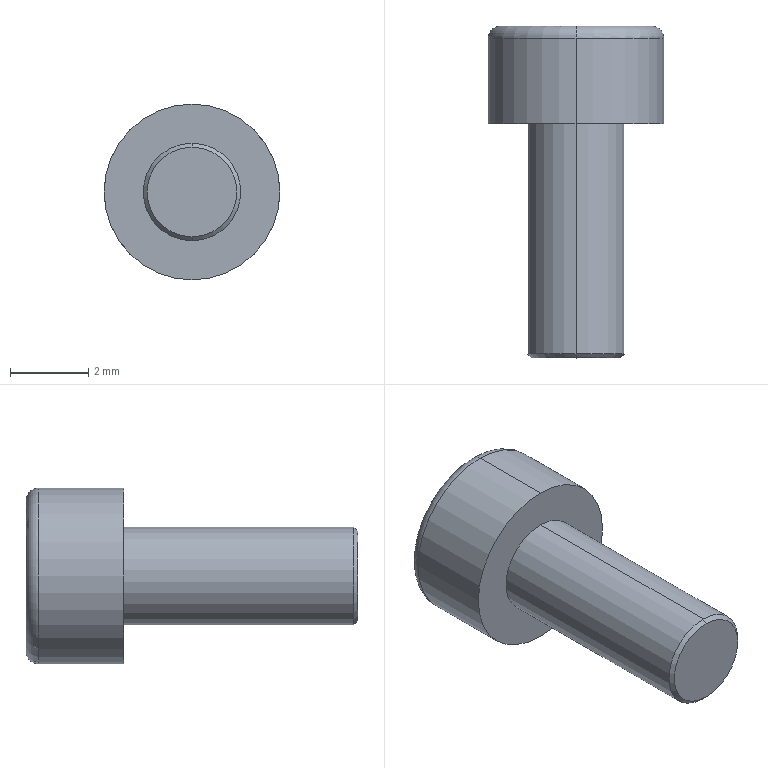Component | SolidWorks | hexagon socket head cap screws gb-1 | 1 solid | 25 faces | box 4.5 x 8.5 x 4.5 mm | volume 64 mm3 | plane 15 | cone 4 | cylinder 4 | torus 2 | commonest cylinder face diameters 2.5 x2 4.5 x2
STEP:
#1=COLOUR_RGB('',0.7922,0.8196,0.9333);
#2=FILL_AREA_STYLE_COLOUR('',#1);
#3=FILL_AREA_STYLE('',(#2));
#4=SURFACE_STYLE_FILL_AREA(#3);
#5=SURFACE_SIDE_STYLE('',(#4));
#6=SURFACE_STYLE_USAGE(.BOTH.,#5);
#7=PRESENTATION_STYLE_ASSIGNMENT((#6));
#8=CARTESIAN_POINT('',(-0.8485,0.2798,5.9));
#9=VERTEX_POINT('',#8);
#10=CARTESIAN_POINT('',(-0.8485,0.2798,5.991));
#11=VERTEX_POINT('',#10);
#12=CARTESIAN_POINT('',(-0.8485,0.2798,5.945));
#13=DIRECTION('',(0.,-1.,0.));
#14=DIRECTION('',(0.,0.,-1.));
#15=AXIS2_PLACEMENT_3D('',#12,#13,#14);
#16=CIRCLE('',#15,0.04528);
#17=EDGE_CURVE('',#9,#11,#16,.T.);
#18=ORIENTED_EDGE('',*,*,#17,.F.);
#19=CARTESIAN_POINT('',(-0.8485,0.2837,5.896));
#20=VERTEX_POINT('',#19);
#21=CARTESIAN_POINT('',(-0.8485,0.2798,5.9));
#22=DIRECTION('',(0.,0.7071,-0.7071));
#23=VECTOR('',#22,39.37);
#24=LINE('',#21,#23);
#25=EDGE_CURVE('',#9,#20,#24,.T.);
#26=ORIENTED_EDGE('',*,*,#25,.T.);
#27=CARTESIAN_POINT('',(-0.8485,0.2837,5.994));
#28=VERTEX_POINT('',#27);
#29=CARTESIAN_POINT('',(-0.8485,0.2837,5.945));
#30=DIRECTION('',(0.,1.,0.));
#31=DIRECTION('',(0.,0.,-1.));
#32=AXIS2_PLACEMENT_3D('',#29,#30,#31);
#33=CIRCLE('',#32,0.04921);
#34=EDGE_CURVE('',#28,#20,#33,.T.);
#35=ORIENTED_EDGE('',*,*,#34,.F.);
#36=CARTESIAN_POINT('',(-0.8485,0.2798,5.991));
#37=DIRECTION('',(0.,0.7071,0.7071));
#38=VECTOR('',#37,39.37);
#39=LINE('',#36,#38);
#40=EDGE_CURVE('',#11,#28,#39,.T.);
#41=ORIENTED_EDGE('',*,*,#40,.F.);
#42=EDGE_LOOP('',(#18,#26,#35,#41));
#43=FACE_OUTER_BOUND('',#42,.T.);
#44=CARTESIAN_POINT('',(-0.8485,0.2798,5.945));
#45=DIRECTION('',(0.,1.,0.));
#46=DIRECTION('',(0.,0.,1.));
#47=AXIS2_PLACEMENT_3D('',#44,#45,#46);
#48=CONICAL_SURFACE('',#47,0.04528,0.7854);
#49=ADVANCED_FACE('',(#43),#48,.T.);
#50=CARTESIAN_POINT('',(-0.8485,0.6144,6.022));
#51=VERTEX_POINT('',#50);
#52=CARTESIAN_POINT('',(-0.8485,0.6144,5.869));
#53=VERTEX_POINT('',#52);
#54=CARTESIAN_POINT('',(-0.8485,0.6144,5.945));
#55=DIRECTION('',(0.,1.,0.));
#56=DIRECTION('',(0.,0.,-1.));
#57=AXIS2_PLACEMENT_3D('',#54,#55,#56);
#58=CIRCLE('',#57,0.07628);
#59=EDGE_CURVE('',#51,#53,#58,.T.);
#60=ORIENTED_EDGE('',*,*,#59,.F.);
#61=CARTESIAN_POINT('',(-0.8485,0.6021,6.034));
#62=VERTEX_POINT('',#61);
#63=CARTESIAN_POINT('',(-0.8485,0.6021,6.022));
#64=DIRECTION('',(1.,0.,-0.));
#65=DIRECTION('',(0.,0.,-1.));
#66=AXIS2_PLACEMENT_3D('',#63,#64,#65);
#67=CIRCLE('',#66,0.0123);
#68=EDGE_CURVE('',#51,#62,#67,.T.);
#69=ORIENTED_EDGE('',*,*,#68,.T.);
#70=CARTESIAN_POINT('',(-0.8485,0.6021,5.857));
#71=VERTEX_POINT('',#70);
#72=CARTESIAN_POINT('',(-0.8485,0.6021,5.945));
#73=DIRECTION('',(0.,-1.,0.));
#74=DIRECTION('',(0.,0.,-1.));
#75=AXIS2_PLACEMENT_3D('',#72,#73,#74);
#76=CIRCLE('',#75,0.08858);
#77=EDGE_CURVE('',#71,#62,#76,.T.);
#78=ORIENTED_EDGE('',*,*,#77,.F.);
#79=CARTESIAN_POINT('',(-0.8485,0.6021,5.869));
#80=DIRECTION('',(-1.,0.,0.));
#81=DIRECTION('',(0.,0.,1.));
#82=AXIS2_PLACEMENT_3D('',#79,#80,#81);
#83=CIRCLE('',#82,0.0123);
#84=EDGE_CURVE('',#53,#71,#83,.T.);
#85=ORIENTED_EDGE('',*,*,#84,.F.);
#86=EDGE_LOOP('',(#60,#69,#78,#85));
#87=FACE_OUTER_BOUND('',#86,.T.);
#88=CARTESIAN_POINT('',(-0.8485,0.6021,5.945));
#89=DIRECTION('',(0.,-1.,0.));
#90=DIRECTION('',(0.,0.,-1.));
#91=AXIS2_PLACEMENT_3D('',#88,#89,#90);
#92=TOROIDAL_SURFACE('',#91,0.07628,0.0123);
#93=ADVANCED_FACE('',(#87),#92,.T.);
#94=CARTESIAN_POINT('',(-0.8485,0.5484,5.945));
#95=VERTEX_POINT('',#94);
#96=CARTESIAN_POINT('',(-0.8485,0.5711,5.985));
#97=VERTEX_POINT('',#96);
#98=CARTESIAN_POINT('',(-0.8485,0.5711,5.985));
#99=DIRECTION('',(0.,0.5,0.866));
#100=VECTOR('',#99,39.37);
#101=LINE('',#98,#100);
#102=EDGE_CURVE('',#95,#97,#101,.T.);
#103=ORIENTED_EDGE('',*,*,#102,.F.);
#104=CARTESIAN_POINT('',(-0.8485,0.5711,5.906));
#105=VERTEX_POINT('',#104);
#106=CARTESIAN_POINT('',(-0.8485,0.5711,5.906));
#107=DIRECTION('',(0.,0.5,-0.866));
#108=VECTOR('',#107,39.37);
#109=LINE('',#106,#108);
#110=EDGE_CURVE('',#95,#105,#109,.T.);
#111=ORIENTED_EDGE('',*,*,#110,.T.);
#112=CARTESIAN_POINT('',(-0.8682,0.5711,5.911));
#113=VERTEX_POINT('',#112);
#114=CARTESIAN_POINT('',(-0.8485,0.5711,5.945));
#115=DIRECTION('',(0.,1.,0.));
#116=DIRECTION('',(0.,0.,-1.));
#117=AXIS2_PLACEMENT_3D('',#114,#115,#116);
#118=CIRCLE('',#117,0.03937);
#119=EDGE_CURVE('',#105,#113,#118,.T.);
#120=ORIENTED_EDGE('',*,*,#119,.T.);
#121=CARTESIAN_POINT('',(-0.8879,0.5711,5.945));
#122=VERTEX_POINT('',#121);
#123=CARTESIAN_POINT('',(-0.8485,0.5711,5.945));
#124=DIRECTION('',(0.,1.,0.));
#125=DIRECTION('',(0.,0.,-1.));
#126=AXIS2_PLACEMENT_3D('',#123,#124,#125);
#127=CIRCLE('',#126,0.03937);
#128=EDGE_CURVE('',#113,#122,#127,.T.);
#129=ORIENTED_EDGE('',*,*,#128,.T.);
#130=CARTESIAN_POINT('',(-0.8682,0.5711,5.979));
#131=VERTEX_POINT('',#130);
#132=CARTESIAN_POINT('',(-0.8485,0.5711,5.945));
#133=DIRECTION('',(0.,1.,0.));
#134=DIRECTION('',(-0.,0.,-1.));
#135=AXIS2_PLACEMENT_3D('',#132,#133,#134);
#136=CIRCLE('',#135,0.03937);
#137=EDGE_CURVE('',#122,#131,#136,.T.);
#138=ORIENTED_EDGE('',*,*,#137,.T.);
#139=CARTESIAN_POINT('',(-0.8485,0.5711,5.945));
#140=DIRECTION('',(0.,1.,0.));
#141=DIRECTION('',(0.,0.,-1.));
#142=AXIS2_PLACEMENT_3D('',#139,#140,#141);
#143=CIRCLE('',#142,0.03937);
#144=EDGE_CURVE('',#131,#97,#143,.T.);
#145=ORIENTED_EDGE('',*,*,#144,.T.);
#146=EDGE_LOOP('',(#103,#111,#120,#129,#138,#145));
#147=FACE_OUTER_BOUND('',#146,.T.);
#148=CARTESIAN_POINT('',(-0.8485,0.5711,5.945));
#149=DIRECTION('',(0.,1.,0.));
#150=DIRECTION('',(0.,0.,1.));
#151=AXIS2_PLACEMENT_3D('',#148,#149,#150);
#152=CONICAL_SURFACE('',#151,0.03937,1.047);
#153=ADVANCED_FACE('',(#147),#152,.F.);
#154=ORIENTED_EDGE('',*,*,#34,.T.);
#155=CARTESIAN_POINT('',(-0.8485,0.516,5.896));
#156=VERTEX_POINT('',#155);
#157=CARTESIAN_POINT('',(-0.8485,0.2798,5.896));
#158=DIRECTION('',(0.,1.,0.));
#159=VECTOR('',#158,39.37);
#160=LINE('',#157,#159);
#161=EDGE_CURVE('',#20,#156,#160,.T.);
#162=ORIENTED_EDGE('',*,*,#161,.T.);
#163=CARTESIAN_POINT('',(-0.8485,0.516,5.994));
#164=VERTEX_POINT('',#163);
#165=CARTESIAN_POINT('',(-0.8485,0.516,5.945));
#166=DIRECTION('',(0.,-1.,0.));
#167=DIRECTION('',(0.,0.,-1.));
#168=AXIS2_PLACEMENT_3D('',#165,#166,#167);
#169=CIRCLE('',#168,0.04921);
#170=EDGE_CURVE('',#156,#164,#169,.T.);
#171=ORIENTED_EDGE('',*,*,#170,.T.);
#172=CARTESIAN_POINT('',(-0.8485,0.2798,5.994));
#173=DIRECTION('',(0.,1.,0.));
#174=VECTOR('',#173,39.37);
#175=LINE('',#172,#174);
#176=EDGE_CURVE('',#28,#164,#175,.T.);
#177=ORIENTED_EDGE('',*,*,#176,.F.);
#178=EDGE_LOOP('',(#154,#162,#171,#177));
#179=FACE_OUTER_BOUND('',#178,.T.);
#180=CARTESIAN_POINT('',(-0.8485,0.2798,5.945));
#181=DIRECTION('',(0.,1.,0.));
#182=DIRECTION('',(0.,0.,1.));
#183=AXIS2_PLACEMENT_3D('',#180,#181,#182);
#184=CYLINDRICAL_SURFACE('',#183,0.04921);
#185=ADVANCED_FACE('',(#179),#184,.T.);
#186=CARTESIAN_POINT('',(-0.8485,0.516,5.857));
#187=VERTEX_POINT('',#186);
#188=CARTESIAN_POINT('',(-0.8485,0.516,6.034));
#189=VERTEX_POINT('',#188);
#190=CARTESIAN_POINT('',(-0.8485,0.516,5.945));
#191=DIRECTION('',(0.,-1.,0.));
#192=DIRECTION('',(0.,0.,-1.));
#193=AXIS2_PLACEMENT_3D('',#190,#191,#192);
#194=CIRCLE('',#193,0.08858);
#195=EDGE_CURVE('',#187,#189,#194,.T.);
#196=ORIENTED_EDGE('',*,*,#195,.F.);
#197=CARTESIAN_POINT('',(-0.8485,0.516,5.857));
#198=DIRECTION('',(0.,1.,0.));
#199=VECTOR('',#198,39.37);
#200=LINE('',#197,#199);
#201=EDGE_CURVE('',#187,#71,#200,.T.);
#202=ORIENTED_EDGE('',*,*,#201,.T.);
#203=ORIENTED_EDGE('',*,*,#77,.T.);
#204=CARTESIAN_POINT('',(-0.8485,0.516,6.034));
#205=DIRECTION('',(0.,1.,0.));
#206=VECTOR('',#205,39.37);
#207=LINE('',#204,#206);
#208=EDGE_CURVE('',#189,#62,#207,.T.);
#209=ORIENTED_EDGE('',*,*,#208,.F.);
#210=EDGE_LOOP('',(#196,#202,#203,#209));
#211=FACE_OUTER_BOUND('',#210,.T.);
#212=CARTESIAN_POINT('',(-0.8485,0.516,5.945));
#213=DIRECTION('',(0.,1.,0.));
#214=DIRECTION('',(0.,0.,1.));
#215=AXIS2_PLACEMENT_3D('',#212,#213,#214);
#216=CYLINDRICAL_SURFACE('',#215,0.08858);
#217=ADVANCED_FACE('',(#211),#216,.T.);
#218=ORIENTED_EDGE('',*,*,#128,.F.);
#219=CARTESIAN_POINT('',(-0.8879,0.5711,5.923));
#220=VERTEX_POINT('',#219);
#221=CARTESIAN_POINT('',(-0.8879,0.5711,5.923));
#222=DIRECTION('',(0.866,0.,-0.5));
#223=VECTOR('',#222,39.37);
#224=LINE('',#221,#223);
#225=EDGE_CURVE('',#220,#113,#224,.T.);
#226=ORIENTED_EDGE('',*,*,#225,.F.);
#227=CARTESIAN_POINT('',(-0.8879,0.5711,5.968));
#228=DIRECTION('',(0.,0.,-1.));
#229=VECTOR('',#228,39.37);
#230=LINE('',#227,#229);
#231=EDGE_CURVE('',#122,#220,#230,.T.);
#232=ORIENTED_EDGE('',*,*,#231,.F.);
#233=EDGE_LOOP('',(#218,#226,#232));
#234=FACE_OUTER_BOUND('',#233,.T.);
#235=CARTESIAN_POINT('',(-0.8485,0.5711,5.9));
#236=DIRECTION('',(0.,-1.,0.));
#237=DIRECTION('',(0.,0.,-1.));
#238=AXIS2_PLACEMENT_3D('',#235,#236,#237);
#239=PLANE('',#238);
#240=ADVANCED_FACE('',(#234),#239,.F.);
#241=ORIENTED_EDGE('',*,*,#137,.F.);
#242=CARTESIAN_POINT('',(-0.8879,0.5711,5.968));
#243=VERTEX_POINT('',#242);
#244=CARTESIAN_POINT('',(-0.8879,0.5711,5.968));
#245=DIRECTION('',(0.,0.,-1.));
#246=VECTOR('',#245,39.37);
#247=LINE('',#244,#246);
#248=EDGE_CURVE('',#243,#122,#247,.T.);
#249=ORIENTED_EDGE('',*,*,#248,.F.);
#250=CARTESIAN_POINT('',(-0.8485,0.5711,5.991));
#251=DIRECTION('',(-0.866,0.,-0.5));
#252=VECTOR('',#251,39.37);
#253=LINE('',#250,#252);
#254=EDGE_CURVE('',#131,#243,#253,.T.);
#255=ORIENTED_EDGE('',*,*,#254,.F.);
#256=EDGE_LOOP('',(#241,#249,#255));
#257=FACE_OUTER_BOUND('',#256,.T.);
#258=CARTESIAN_POINT('',(-0.8485,0.5711,5.9));
#259=DIRECTION('',(0.,-1.,0.));
#260=DIRECTION('',(0.,0.,-1.));
#261=AXIS2_PLACEMENT_3D('',#258,#259,#260);
#262=PLANE('',#261);
#263=ADVANCED_FACE('',(#257),#262,.F.);
#264=ORIENTED_EDGE('',*,*,#144,.F.);
#265=CARTESIAN_POINT('',(-0.8485,0.5711,5.991));
#266=VERTEX_POINT('',#265);
#267=CARTESIAN_POINT('',(-0.8485,0.5711,5.991));
#268=DIRECTION('',(-0.866,0.,-0.5));
#269=VECTOR('',#268,39.37);
#270=LINE('',#267,#269);
#271=EDGE_CURVE('',#266,#131,#270,.T.);
#272=ORIENTED_EDGE('',*,*,#271,.F.);
#273=CARTESIAN_POINT('',(-0.8288,0.5711,5.979));
#274=VERTEX_POINT('',#273);
#275=CARTESIAN_POINT('',(-0.8092,0.5711,5.968));
#276=DIRECTION('',(-0.866,0.,0.5));
#277=VECTOR('',#276,39.37);
#278=LINE('',#275,#277);
#279=EDGE_CURVE('',#274,#266,#278,.T.);
#280=ORIENTED_EDGE('',*,*,#279,.F.);
#281=CARTESIAN_POINT('',(-0.8485,0.5711,5.945));
#282=DIRECTION('',(0.,1.,0.));
#283=DIRECTION('',(0.,0.,-1.));
#284=AXIS2_PLACEMENT_3D('',#281,#282,#283);
#285=CIRCLE('',#284,0.03937);
#286=EDGE_CURVE('',#97,#274,#285,.T.);
#287=ORIENTED_EDGE('',*,*,#286,.F.);
#288=EDGE_LOOP('',(#264,#272,#280,#287));
#289=FACE_OUTER_BOUND('',#288,.T.);
#290=CARTESIAN_POINT('',(-0.8485,0.5711,5.9));
#291=DIRECTION('',(0.,-1.,0.));
#292=DIRECTION('',(0.,0.,-1.));
#293=AXIS2_PLACEMENT_3D('',#290,#291,#292);
#294=PLANE('',#293);
#295=ADVANCED_FACE('',(#289),#294,.F.);
#296=CARTESIAN_POINT('',(-0.8092,0.5711,5.945));
#297=VERTEX_POINT('',#296);
#298=CARTESIAN_POINT('',(-0.8485,0.5711,5.945));
#299=DIRECTION('',(0.,1.,0.));
#300=DIRECTION('',(0.,0.,-1.));
#301=AXIS2_PLACEMENT_3D('',#298,#299,#300);
#302=CIRCLE('',#301,0.03937);
#303=EDGE_CURVE('',#274,#297,#302,.T.);
#304=ORIENTED_EDGE('',*,*,#303,.F.);
#305=CARTESIAN_POINT('',(-0.8092,0.5711,5.968));
#306=VERTEX_POINT('',#305);
#307=CARTESIAN_POINT('',(-0.8092,0.5711,5.968));
#308=DIRECTION('',(-0.866,0.,0.5));
#309=VECTOR('',#308,39.37);
#310=LINE('',#307,#309);
#311=EDGE_CURVE('',#306,#274,#310,.T.);
#312=ORIENTED_EDGE('',*,*,#311,.F.);
#313=CARTESIAN_POINT('',(-0.8092,0.5711,5.923));
#314=DIRECTION('',(0.,0.,1.));
#315=VECTOR('',#314,39.37);
#316=LINE('',#313,#315);
#317=EDGE_CURVE('',#297,#306,#316,.T.);
#318=ORIENTED_EDGE('',*,*,#317,.F.);
#319=EDGE_LOOP('',(#304,#312,#318));
#320=FACE_OUTER_BOUND('',#319,.T.);
#321=CARTESIAN_POINT('',(-0.8485,0.5711,5.9));
#322=DIRECTION('',(0.,-1.,0.));
#323=DIRECTION('',(0.,0.,-1.));
#324=AXIS2_PLACEMENT_3D('',#321,#322,#323);
#325=PLANE('',#324);
#326=ADVANCED_FACE('',(#320),#325,.F.);
#327=CARTESIAN_POINT('',(-0.8288,0.5711,5.911));
#328=VERTEX_POINT('',#327);
#329=CARTESIAN_POINT('',(-0.8485,0.5711,5.945));
#330=DIRECTION('',(0.,-1.,0.));
#331=DIRECTION('',(0.,0.,-1.));
#332=AXIS2_PLACEMENT_3D('',#329,#330,#331);
#333=CIRCLE('',#332,0.03937);
#334=EDGE_CURVE('',#328,#297,#333,.T.);
#335=ORIENTED_EDGE('',*,*,#334,.T.);
#336=CARTESIAN_POINT('',(-0.8092,0.5711,5.923));
#337=VERTEX_POINT('',#336);
#338=CARTESIAN_POINT('',(-0.8092,0.5711,5.923));
#339=DIRECTION('',(0.,0.,1.));
#340=VECTOR('',#339,39.37);
#341=LINE('',#338,#340);
#342=EDGE_CURVE('',#337,#297,#341,.T.);
#343=ORIENTED_EDGE('',*,*,#342,.F.);
#344=CARTESIAN_POINT('',(-0.8485,0.5711,5.9));
#345=DIRECTION('',(0.866,0.,0.5));
#346=VECTOR('',#345,39.37);
#347=LINE('',#344,#346);
#348=EDGE_CURVE('',#328,#337,#347,.T.);
#349=ORIENTED_EDGE('',*,*,#348,.F.);
#350=EDGE_LOOP('',(#335,#343,#349));
#351=FACE_OUTER_BOUND('',#350,.T.);
#352=CARTESIAN_POINT('',(-0.8485,0.5711,5.9));
#353=DIRECTION('',(0.,-1.,0.));
#354=DIRECTION('',(0.,0.,-1.));
#355=AXIS2_PLACEMENT_3D('',#352,#353,#354);
#356=PLANE('',#355);
#357=ADVANCED_FACE('',(#351),#356,.F.);
#358=CARTESIAN_POINT('',(-0.8485,0.5711,5.945));
#359=DIRECTION('',(0.,1.,0.));
#360=DIRECTION('',(-0.,0.,-1.));
#361=AXIS2_PLACEMENT_3D('',#358,#359,#360);
#362=CIRCLE('',#361,0.03937);
#363=EDGE_CURVE('',#328,#105,#362,.T.);
#364=ORIENTED_EDGE('',*,*,#363,.F.);
#365=CARTESIAN_POINT('',(-0.8485,0.5711,5.9));
#366=VERTEX_POINT('',#365);
#367=CARTESIAN_POINT('',(-0.8485,0.5711,5.9));
#368=DIRECTION('',(0.866,0.,0.5));
#369=VECTOR('',#368,39.37);
#370=LINE('',#367,#369);
#371=EDGE_CURVE('',#366,#328,#370,.T.);
#372=ORIENTED_EDGE('',*,*,#371,.F.);
#373=CARTESIAN_POINT('',(-0.8879,0.5711,5.923));
#374=DIRECTION('',(0.866,0.,-0.5));
#375=VECTOR('',#374,39.37);
#376=LINE('',#373,#375);
#377=EDGE_CURVE('',#113,#366,#376,.T.);
#378=ORIENTED_EDGE('',*,*,#377,.F.);
#379=ORIENTED_EDGE('',*,*,#119,.F.);
#380=EDGE_LOOP('',(#364,#372,#378,#379));
#381=FACE_OUTER_BOUND('',#380,.T.);
#382=CARTESIAN_POINT('',(-0.8485,0.5711,5.9));
#383=DIRECTION('',(0.,-1.,0.));
#384=DIRECTION('',(0.,0.,-1.));
#385=AXIS2_PLACEMENT_3D('',#382,#383,#384);
#386=PLANE('',#385);
#387=ADVANCED_FACE('',(#381),#386,.F.);
#388=CARTESIAN_POINT('',(-0.8485,0.6144,5.945));
#389=DIRECTION('',(0.,1.,0.));
#390=DIRECTION('',(0.,0.,-1.));
#391=AXIS2_PLACEMENT_3D('',#388,#389,#390);
#392=CIRCLE('',#391,0.07628);
#393=EDGE_CURVE('',#53,#51,#392,.T.);
#394=ORIENTED_EDGE('',*,*,#393,.T.);
#395=ORIENTED_EDGE('',*,*,#59,.T.);
#396=EDGE_LOOP('',(#394,#395));
#397=FACE_OUTER_BOUND('',#396,.T.);
#398=CARTESIAN_POINT('',(-0.8879,0.6144,5.923));
#399=VERTEX_POINT('',#398);
#400=CARTESIAN_POINT('',(-0.8485,0.6144,5.9));
#401=VERTEX_POINT('',#400);
#402=CARTESIAN_POINT('',(-0.8879,0.6144,5.923));
#403=DIRECTION('',(0.866,0.,-0.5));
#404=VECTOR('',#403,39.37);
#405=LINE('',#402,#404);
#406=EDGE_CURVE('',#399,#401,#405,.T.);
#407=ORIENTED_EDGE('',*,*,#406,.T.);
#408=CARTESIAN_POINT('',(-0.8092,0.6144,5.923));
#409=VERTEX_POINT('',#408);
#410=CARTESIAN_POINT('',(-0.8485,0.6144,5.9));
#411=DIRECTION('',(0.866,0.,0.5));
#412=VECTOR('',#411,39.37);
#413=LINE('',#410,#412);
#414=EDGE_CURVE('',#401,#409,#413,.T.);
#415=ORIENTED_EDGE('',*,*,#414,.T.);
#416=CARTESIAN_POINT('',(-0.8092,0.6144,5.968));
#417=VERTEX_POINT('',#416);
#418=CARTESIAN_POINT('',(-0.8092,0.6144,5.923));
#419=DIRECTION('',(0.,0.,1.));
#420=VECTOR('',#419,39.37);
#421=LINE('',#418,#420);
#422=EDGE_CURVE('',#409,#417,#421,.T.);
#423=ORIENTED_EDGE('',*,*,#422,.T.);
#424=CARTESIAN_POINT('',(-0.8485,0.6144,5.991));
#425=VERTEX_POINT('',#424);
#426=CARTESIAN_POINT('',(-0.8092,0.6144,5.968));
#427=DIRECTION('',(-0.866,0.,0.5));
#428=VECTOR('',#427,39.37);
#429=LINE('',#426,#428);
#430=EDGE_CURVE('',#417,#425,#429,.T.);
#431=ORIENTED_EDGE('',*,*,#430,.T.);
#432=CARTESIAN_POINT('',(-0.8879,0.6144,5.968));
#433=VERTEX_POINT('',#432);
#434=CARTESIAN_POINT('',(-0.8485,0.6144,5.991));
#435=DIRECTION('',(-0.866,0.,-0.5));
#436=VECTOR('',#435,39.37);
#437=LINE('',#434,#436);
#438=EDGE_CURVE('',#425,#433,#437,.T.);
#439=ORIENTED_EDGE('',*,*,#438,.T.);
#440=CARTESIAN_POINT('',(-0.8879,0.6144,5.968));
#441=DIRECTION('',(0.,0.,-1.));
#442=VECTOR('',#441,39.37);
#443=LINE('',#440,#442);
#444=EDGE_CURVE('',#433,#399,#443,.T.);
#445=ORIENTED_EDGE('',*,*,#444,.T.);
#446=EDGE_LOOP('',(#407,#415,#423,#431,#439,#445));
#447=FACE_BOUND('',#446,.T.);
#448=CARTESIAN_POINT('',(-0.8485,0.6144,5.945));
#449=DIRECTION('',(0.,-1.,0.));
#450=DIRECTION('',(0.,0.,-1.));
#451=AXIS2_PLACEMENT_3D('',#448,#449,#450);
#452=PLANE('',#451);
#453=ADVANCED_FACE('',(#397,#447),#452,.F.);
#454=CARTESIAN_POINT('',(-0.8485,0.516,5.945));
#455=DIRECTION('',(0.,-1.,0.));
#456=DIRECTION('',(0.,0.,-1.));
#457=AXIS2_PLACEMENT_3D('',#454,#455,#456);
#458=CIRCLE('',#457,0.08858);
#459=EDGE_CURVE('',#189,#187,#458,.T.);
#460=ORIENTED_EDGE('',*,*,#459,.T.);
#461=ORIENTED_EDGE('',*,*,#195,.T.);
#462=EDGE_LOOP('',(#460,#461));
#463=FACE_OUTER_BOUND('',#462,.T.);
#464=CARTESIAN_POINT('',(-0.8485,0.516,5.945));
#465=DIRECTION('',(0.,-1.,0.));
#466=DIRECTION('',(0.,0.,-1.));
#467=AXIS2_PLACEMENT_3D('',#464,#465,#466);
#468=CIRCLE('',#467,0.04921);
#469=EDGE_CURVE('',#164,#156,#468,.T.);
#470=ORIENTED_EDGE('',*,*,#469,.F.);
#471=ORIENTED_EDGE('',*,*,#170,.F.);
#472=EDGE_LOOP('',(#470,#471));
#473=FACE_BOUND('',#472,.T.);
#474=CARTESIAN_POINT('',(-0.8485,0.516,5.945));
#475=DIRECTION('',(0.,-1.,0.));
#476=DIRECTION('',(0.,0.,-1.));
#477=AXIS2_PLACEMENT_3D('',#474,#475,#476);
#478=PLANE('',#477);
#479=ADVANCED_FACE('',(#463,#473),#478,.T.);
#480=ORIENTED_EDGE('',*,*,#201,.F.);
#481=ORIENTED_EDGE('',*,*,#459,.F.);
#482=ORIENTED_EDGE('',*,*,#208,.T.);
#483=CARTESIAN_POINT('',(-0.8485,0.6021,5.945));
#484=DIRECTION('',(0.,-1.,0.));
#485=DIRECTION('',(0.,0.,-1.));
#486=AXIS2_PLACEMENT_3D('',#483,#484,#485);
#487=CIRCLE('',#486,0.08858);
#488=EDGE_CURVE('',#62,#71,#487,.T.);
#489=ORIENTED_EDGE('',*,*,#488,.T.);
#490=EDGE_LOOP('',(#480,#481,#482,#489));
#491=FACE_OUTER_BOUND('',#490,.T.);
#492=CARTESIAN_POINT('',(-0.8485,0.516,5.945));
#493=DIRECTION('',(0.,1.,0.));
#494=DIRECTION('',(0.,0.,1.));
#495=AXIS2_PLACEMENT_3D('',#492,#493,#494);
#496=CYLINDRICAL_SURFACE('',#495,0.08858);
#497=ADVANCED_FACE('',(#491),#496,.T.);
#498=ORIENTED_EDGE('',*,*,#161,.F.);
#499=CARTESIAN_POINT('',(-0.8485,0.2837,5.945));
#500=DIRECTION('',(0.,1.,0.));
#501=DIRECTION('',(0.,0.,-1.));
#502=AXIS2_PLACEMENT_3D('',#499,#500,#501);
#503=CIRCLE('',#502,0.04921);
#504=EDGE_CURVE('',#20,#28,#503,.T.);
#505=ORIENTED_EDGE('',*,*,#504,.T.);
#506=ORIENTED_EDGE('',*,*,#176,.T.);
#507=ORIENTED_EDGE('',*,*,#469,.T.);
#508=EDGE_LOOP('',(#498,#505,#506,#507));
#509=FACE_OUTER_BOUND('',#508,.T.);
#510=CARTESIAN_POINT('',(-0.8485,0.2798,5.945));
#511=DIRECTION('',(0.,1.,0.));
#512=DIRECTION('',(0.,0.,1.));
#513=AXIS2_PLACEMENT_3D('',#510,#511,#512);
#514=CYLINDRICAL_SURFACE('',#513,0.04921);
#515=ADVANCED_FACE('',(#509),#514,.T.);
#516=CARTESIAN_POINT('',(-0.8485,0.2798,5.945));
#517=DIRECTION('',(0.,-1.,0.));
#518=DIRECTION('',(0.,0.,-1.));
#519=AXIS2_PLACEMENT_3D('',#516,#517,#518);
#520=CIRCLE('',#519,0.04528);
#521=EDGE_CURVE('',#11,#9,#520,.T.);
#522=ORIENTED_EDGE('',*,*,#521,.T.);
#523=ORIENTED_EDGE('',*,*,#17,.T.);
#524=EDGE_LOOP('',(#522,#523));
#525=FACE_OUTER_BOUND('',#524,.T.);
#526=CARTESIAN_POINT('',(-0.8485,0.2798,5.945));
#527=DIRECTION('',(0.,-1.,0.));
#528=DIRECTION('',(0.,0.,-1.));
#529=AXIS2_PLACEMENT_3D('',#526,#527,#528);
#530=PLANE('',#529);
#531=ADVANCED_FACE('',(#525),#530,.T.);
#532=ORIENTED_EDGE('',*,*,#406,.F.);
#533=CARTESIAN_POINT('',(-0.8879,0.5711,5.923));
#534=DIRECTION('',(0.,1.,0.));
#535=VECTOR('',#534,39.37);
#536=LINE('',#533,#535);
#537=EDGE_CURVE('',#220,#399,#536,.T.);
#538=ORIENTED_EDGE('',*,*,#537,.F.);
#539=ORIENTED_EDGE('',*,*,#225,.T.);
#540=ORIENTED_EDGE('',*,*,#377,.T.);
#541=CARTESIAN_POINT('',(-0.8485,0.5711,5.9));
#542=DIRECTION('',(0.,1.,0.));
#543=VECTOR('',#542,39.37);
#544=LINE('',#541,#543);
#545=EDGE_CURVE('',#366,#401,#544,.T.);
#546=ORIENTED_EDGE('',*,*,#545,.T.);
#547=EDGE_LOOP('',(#532,#538,#539,#540,#546));
#548=FACE_OUTER_BOUND('',#547,.T.);
#549=CARTESIAN_POINT('',(-0.8879,0.5711,5.923));
#550=DIRECTION('',(0.5,0.,0.866));
#551=DIRECTION('',(-0.866,0.,0.5));
#552=AXIS2_PLACEMENT_3D('',#549,#550,#551);
#553=PLANE('',#552);
#554=ADVANCED_FACE('',(#548),#553,.T.);
#555=ORIENTED_EDGE('',*,*,#414,.F.);
#556=ORIENTED_EDGE('',*,*,#545,.F.);
#557=ORIENTED_EDGE('',*,*,#371,.T.);
#558=ORIENTED_EDGE('',*,*,#348,.T.);
#559=CARTESIAN_POINT('',(-0.8092,0.5711,5.923));
#560=DIRECTION('',(0.,1.,0.));
#561=VECTOR('',#560,39.37);
#562=LINE('',#559,#561);
#563=EDGE_CURVE('',#337,#409,#562,.T.);
#564=ORIENTED_EDGE('',*,*,#563,.T.);
#565=EDGE_LOOP('',(#555,#556,#557,#558,#564));
#566=FACE_OUTER_BOUND('',#565,.T.);
#567=CARTESIAN_POINT('',(-0.8485,0.5711,5.9));
#568=DIRECTION('',(-0.5,0.,0.866));
#569=DIRECTION('',(-0.866,0.,-0.5));
#570=AXIS2_PLACEMENT_3D('',#567,#568,#569);
#571=PLANE('',#570);
#572=ADVANCED_FACE('',(#566),#571,.T.);
#573=ORIENTED_EDGE('',*,*,#422,.F.);
#574=ORIENTED_EDGE('',*,*,#563,.F.);
#575=ORIENTED_EDGE('',*,*,#342,.T.);
#576=ORIENTED_EDGE('',*,*,#317,.T.);
#577=CARTESIAN_POINT('',(-0.8092,0.5711,5.968));
#578=DIRECTION('',(0.,1.,0.));
#579=VECTOR('',#578,39.37);
#580=LINE('',#577,#579);
#581=EDGE_CURVE('',#306,#417,#580,.T.);
#582=ORIENTED_EDGE('',*,*,#581,.T.);
#583=EDGE_LOOP('',(#573,#574,#575,#576,#582));
#584=FACE_OUTER_BOUND('',#583,.T.);
#585=CARTESIAN_POINT('',(-0.8092,0.5711,5.923));
#586=DIRECTION('',(-1.,0.,0.));
#587=DIRECTION('',(0.,0.,-1.));
#588=AXIS2_PLACEMENT_3D('',#585,#586,#587);
#589=PLANE('',#588);
#590=ADVANCED_FACE('',(#584),#589,.T.);
#591=ORIENTED_EDGE('',*,*,#430,.F.);
#592=ORIENTED_EDGE('',*,*,#581,.F.);
#593=ORIENTED_EDGE('',*,*,#311,.T.);
#594=ORIENTED_EDGE('',*,*,#279,.T.);
#595=CARTESIAN_POINT('',(-0.8485,0.5711,5.991));
#596=DIRECTION('',(0.,1.,0.));
#597=VECTOR('',#596,39.37);
#598=LINE('',#595,#597);
#599=EDGE_CURVE('',#266,#425,#598,.T.);
#600=ORIENTED_EDGE('',*,*,#599,.T.);
#601=EDGE_LOOP('',(#591,#592,#593,#594,#600));
#602=FACE_OUTER_BOUND('',#601,.T.);
#603=CARTESIAN_POINT('',(-0.8092,0.5711,5.968));
#604=DIRECTION('',(-0.5,0.,-0.866));
#605=DIRECTION('',(0.866,0.,-0.5));
#606=AXIS2_PLACEMENT_3D('',#603,#604,#605);
#607=PLANE('',#606);
#608=ADVANCED_FACE('',(#602),#607,.T.);
#609=ORIENTED_EDGE('',*,*,#438,.F.);
#610=ORIENTED_EDGE('',*,*,#599,.F.);
#611=ORIENTED_EDGE('',*,*,#271,.T.);
#612=ORIENTED_EDGE('',*,*,#254,.T.);
#613=CARTESIAN_POINT('',(-0.8879,0.5711,5.968));
#614=DIRECTION('',(0.,1.,0.));
#615=VECTOR('',#614,39.37);
#616=LINE('',#613,#615);
#617=EDGE_CURVE('',#243,#433,#616,.T.);
#618=ORIENTED_EDGE('',*,*,#617,.T.);
#619=EDGE_LOOP('',(#609,#610,#611,#612,#618));
#620=FACE_OUTER_BOUND('',#619,.T.);
#621=CARTESIAN_POINT('',(-0.8485,0.5711,5.991));
#622=DIRECTION('',(0.5,0.,-0.866));
#623=DIRECTION('',(0.866,0.,0.5));
#624=AXIS2_PLACEMENT_3D('',#621,#622,#623);
#625=PLANE('',#624);
#626=ADVANCED_FACE('',(#620),#625,.T.);
#627=ORIENTED_EDGE('',*,*,#444,.F.);
#628=ORIENTED_EDGE('',*,*,#617,.F.);
#629=ORIENTED_EDGE('',*,*,#248,.T.);
#630=ORIENTED_EDGE('',*,*,#231,.T.);
#631=ORIENTED_EDGE('',*,*,#537,.T.);
#632=EDGE_LOOP('',(#627,#628,#629,#630,#631));
#633=FACE_OUTER_BOUND('',#632,.T.);
#634=CARTESIAN_POINT('',(-0.8879,0.5711,5.968));
#635=DIRECTION('',(1.,0.,0.));
#636=DIRECTION('',(-0.,0.,1.));
#637=AXIS2_PLACEMENT_3D('',#634,#635,#636);
#638=PLANE('',#637);
#639=ADVANCED_FACE('',(#633),#638,.T.);
#640=ORIENTED_EDGE('',*,*,#110,.F.);
#641=ORIENTED_EDGE('',*,*,#102,.T.);
#642=ORIENTED_EDGE('',*,*,#286,.T.);
#643=ORIENTED_EDGE('',*,*,#303,.T.);
#644=ORIENTED_EDGE('',*,*,#334,.F.);
#645=ORIENTED_EDGE('',*,*,#363,.T.);
#646=EDGE_LOOP('',(#640,#641,#642,#643,#644,#645));
#647=FACE_OUTER_BOUND('',#646,.T.);
#648=CARTESIAN_POINT('',(-0.8485,0.5711,5.945));
#649=DIRECTION('',(0.,1.,0.));
#650=DIRECTION('',(0.,0.,1.));
#651=AXIS2_PLACEMENT_3D('',#648,#649,#650);
#652=CONICAL_SURFACE('',#651,0.03937,1.047);
#653=ADVANCED_FACE('',(#647),#652,.F.);
#654=ORIENTED_EDGE('',*,*,#68,.F.);
#655=ORIENTED_EDGE('',*,*,#393,.F.);
#656=ORIENTED_EDGE('',*,*,#84,.T.);
#657=ORIENTED_EDGE('',*,*,#488,.F.);
#658=EDGE_LOOP('',(#654,#655,#656,#657));
#659=FACE_OUTER_BOUND('',#658,.T.);
#660=CARTESIAN_POINT('',(-0.8485,0.6021,5.945));
#661=DIRECTION('',(0.,-1.,0.));
#662=DIRECTION('',(0.,0.,-1.));
#663=AXIS2_PLACEMENT_3D('',#660,#661,#662);
#664=TOROIDAL_SURFACE('',#663,0.07628,0.0123);
#665=ADVANCED_FACE('',(#659),#664,.T.);
#666=ORIENTED_EDGE('',*,*,#25,.F.);
#667=ORIENTED_EDGE('',*,*,#521,.F.);
#668=ORIENTED_EDGE('',*,*,#40,.T.);
#669=ORIENTED_EDGE('',*,*,#504,.F.);
#670=EDGE_LOOP('',(#666,#667,#668,#669));
#671=FACE_OUTER_BOUND('',#670,.T.);
#672=CARTESIAN_POINT('',(-0.8485,0.2798,5.945));
#673=DIRECTION('',(0.,1.,0.));
#674=DIRECTION('',(0.,0.,1.));
#675=AXIS2_PLACEMENT_3D('',#672,#673,#674);
#676=CONICAL_SURFACE('',#675,0.04528,0.7854);
#677=ADVANCED_FACE('',(#671),#676,.T.);
#678=CLOSED_SHELL('',(#49,#93,#153,#185,#217,#240,#263,#295,#326,#357,#387,#453,#479,#497,#515,#531,#554,#572,#590,#608,#626,#639,#653,#665,#677));
#679=MANIFOLD_SOLID_BREP('',#678);
#680=STYLED_ITEM('',(#7),#679);
#681=PRESENTATION_LAYER_ASSIGNMENT('','',(#680));
#682=(LENGTH_UNIT()NAMED_UNIT(*)SI_UNIT($,.METRE.));
#683=LENGTH_MEASURE_WITH_UNIT(LENGTH_MEASURE(0.0254),#682);
#684=DIMENSIONAL_EXPONENTS(1.,0.,0.,0.,0.,0.,0.);
#685=(CONVERSION_BASED_UNIT('',#683)LENGTH_UNIT()NAMED_UNIT(#684));
#686=UNCERTAINTY_MEASURE_WITH_UNIT(LENGTH_MEASURE(0.00001),#685,'','');
#687=(NAMED_UNIT(*)PLANE_ANGLE_UNIT()SI_UNIT($,.RADIAN.));
#688=(NAMED_UNIT(*)SI_UNIT($,.STERADIAN.)SOLID_ANGLE_UNIT());
#689=(GEOMETRIC_REPRESENTATION_CONTEXT(3)GLOBAL_UNCERTAINTY_ASSIGNED_CONTEXT((#686))GLOBAL_UNIT_ASSIGNED_CONTEXT((#685,#687,#688))REPRESENTATION_CONTEXT('',''));
#690=MECHANICAL_DESIGN_GEOMETRIC_PRESENTATION_REPRESENTATION('',(#680),#689);
#691=CARTESIAN_POINT('',(0.,0.,0.));
#692=DIRECTION('',(0.,0.,1.));
#693=DIRECTION('',(1.,0.,0.));
#694=AXIS2_PLACEMENT_3D('',#691,#692,#693);
#695=(LENGTH_UNIT()NAMED_UNIT(*)SI_UNIT($,.METRE.));
#696=LENGTH_MEASURE_WITH_UNIT(LENGTH_MEASURE(0.0254),#695);
#697=DIMENSIONAL_EXPONENTS(1.,0.,0.,0.,0.,0.,0.);
#698=(CONVERSION_BASED_UNIT('',#696)LENGTH_UNIT()NAMED_UNIT(#697));
#699=UNCERTAINTY_MEASURE_WITH_UNIT(LENGTH_MEASURE(0.00001),#698,'','');
#700=(NAMED_UNIT(*)PLANE_ANGLE_UNIT()SI_UNIT($,.RADIAN.));
#701=(NAMED_UNIT(*)SI_UNIT($,.STERADIAN.)SOLID_ANGLE_UNIT());
#702=(GEOMETRIC_REPRESENTATION_CONTEXT(3)GLOBAL_UNCERTAINTY_ASSIGNED_CONTEXT((#699))GLOBAL_UNIT_ASSIGNED_CONTEXT((#698,#700,#701))REPRESENTATION_CONTEXT('',''));
#703=ADVANCED_BREP_SHAPE_REPRESENTATION('',(#679,#694),#702);